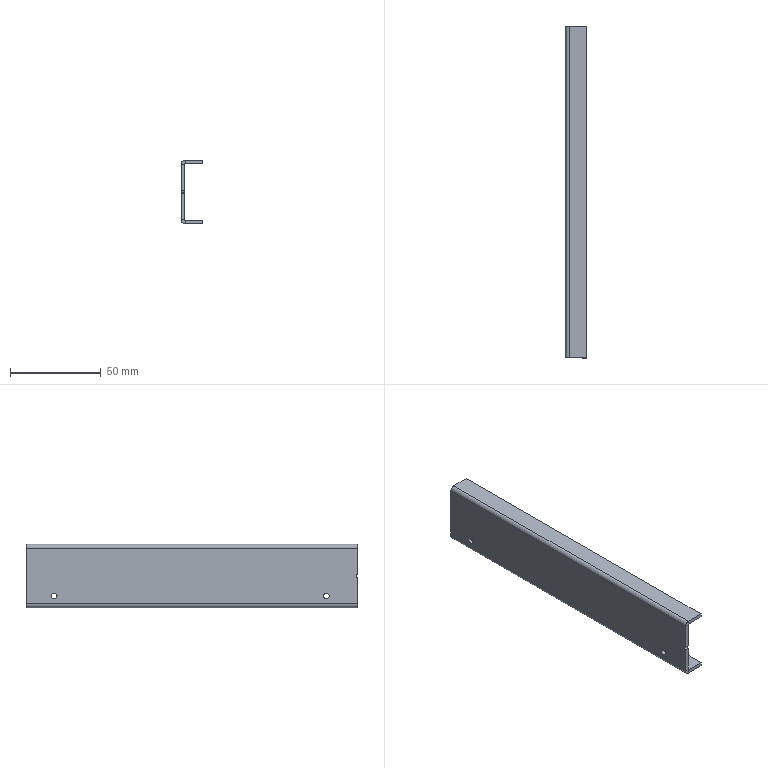Component | SolidWorks | PG50-06(BottomPlateWeldingDrawing)-1_BasePlateWeldment3-A(PG50-05-103-1 | 1 solid | 29 faces | box 12 x 183 x 35 mm | volume 19733 mm3 | plane 19 | cylinder 10 | commonest cylinder face diameters 3.2 x4 2 x2 4.3 x2 0.3 x2 | material AISI 1045 Steel, cold drawn
STEP:
#1=COLOUR_RGB('',0.7922,0.8196,0.9333);
#2=FILL_AREA_STYLE_COLOUR('',#1);
#3=FILL_AREA_STYLE('',(#2));
#4=SURFACE_STYLE_FILL_AREA(#3);
#5=SURFACE_SIDE_STYLE('',(#4));
#6=SURFACE_STYLE_USAGE(.BOTH.,#5);
#7=PRESENTATION_STYLE_ASSIGNMENT((#6));
#8=CARTESIAN_POINT('',(39.678,7.603,-4.154));
#9=VERTEX_POINT('',#8);
#10=CARTESIAN_POINT('',(39.678,7.729,-4.154));
#11=VERTEX_POINT('',#10);
#12=CARTESIAN_POINT('',(39.678,7.666,-4.154));
#13=DIRECTION('',(1.,-0.,0.));
#14=DIRECTION('',(0.,1.,0.));
#15=AXIS2_PLACEMENT_3D('',#12,#13,#14);
#16=CIRCLE('',#15,0.06299);
#17=EDGE_CURVE('',#9,#11,#16,.T.);
#18=ORIENTED_EDGE('',*,*,#17,.F.);
#19=CARTESIAN_POINT('',(39.757,7.603,-4.154));
#20=VERTEX_POINT('',#19);
#21=CARTESIAN_POINT('',(39.678,7.603,-4.154));
#22=DIRECTION('',(1.,-0.,0.));
#23=VECTOR('',#22,39.37);
#24=LINE('',#21,#23);
#25=EDGE_CURVE('',#9,#20,#24,.T.);
#26=ORIENTED_EDGE('',*,*,#25,.T.);
#27=CARTESIAN_POINT('',(39.757,7.729,-4.154));
#28=VERTEX_POINT('',#27);
#29=CARTESIAN_POINT('',(39.757,7.666,-4.154));
#30=DIRECTION('',(1.,-0.,0.));
#31=DIRECTION('',(0.,1.,0.));
#32=AXIS2_PLACEMENT_3D('',#29,#30,#31);
#33=CIRCLE('',#32,0.06299);
#34=EDGE_CURVE('',#20,#28,#33,.T.);
#35=ORIENTED_EDGE('',*,*,#34,.T.);
#36=CARTESIAN_POINT('',(39.678,7.729,-4.154));
#37=DIRECTION('',(1.,-0.,0.));
#38=VECTOR('',#37,39.37);
#39=LINE('',#36,#38);
#40=EDGE_CURVE('',#11,#28,#39,.T.);
#41=ORIENTED_EDGE('',*,*,#40,.F.);
#42=EDGE_LOOP('',(#18,#26,#35,#41));
#43=FACE_OUTER_BOUND('',#42,.T.);
#44=CARTESIAN_POINT('',(39.678,7.666,-4.154));
#45=DIRECTION('',(1.,-0.,0.));
#46=DIRECTION('',(0.,1.,0.));
#47=AXIS2_PLACEMENT_3D('',#44,#45,#46);
#48=CYLINDRICAL_SURFACE('',#47,0.06299);
#49=ADVANCED_FACE('',(#43),#48,.F.);
#50=CARTESIAN_POINT('',(39.678,1.697,-4.154));
#51=VERTEX_POINT('',#50);
#52=CARTESIAN_POINT('',(39.678,1.823,-4.154));
#53=VERTEX_POINT('',#52);
#54=CARTESIAN_POINT('',(39.678,1.76,-4.154));
#55=DIRECTION('',(1.,-0.,0.));
#56=DIRECTION('',(0.,1.,0.));
#57=AXIS2_PLACEMENT_3D('',#54,#55,#56);
#58=CIRCLE('',#57,0.06299);
#59=EDGE_CURVE('',#51,#53,#58,.T.);
#60=ORIENTED_EDGE('',*,*,#59,.F.);
#61=CARTESIAN_POINT('',(39.757,1.697,-4.154));
#62=VERTEX_POINT('',#61);
#63=CARTESIAN_POINT('',(39.678,1.697,-4.154));
#64=DIRECTION('',(1.,-0.,0.));
#65=VECTOR('',#64,39.37);
#66=LINE('',#63,#65);
#67=EDGE_CURVE('',#51,#62,#66,.T.);
#68=ORIENTED_EDGE('',*,*,#67,.T.);
#69=CARTESIAN_POINT('',(39.757,1.823,-4.154));
#70=VERTEX_POINT('',#69);
#71=CARTESIAN_POINT('',(39.757,1.76,-4.154));
#72=DIRECTION('',(1.,-0.,0.));
#73=DIRECTION('',(0.,1.,0.));
#74=AXIS2_PLACEMENT_3D('',#71,#72,#73);
#75=CIRCLE('',#74,0.06299);
#76=EDGE_CURVE('',#62,#70,#75,.T.);
#77=ORIENTED_EDGE('',*,*,#76,.T.);
#78=CARTESIAN_POINT('',(39.678,1.823,-4.154));
#79=DIRECTION('',(1.,-0.,0.));
#80=VECTOR('',#79,39.37);
#81=LINE('',#78,#80);
#82=EDGE_CURVE('',#53,#70,#81,.T.);
#83=ORIENTED_EDGE('',*,*,#82,.F.);
#84=EDGE_LOOP('',(#60,#68,#77,#83));
#85=FACE_OUTER_BOUND('',#84,.T.);
#86=CARTESIAN_POINT('',(39.678,1.76,-4.154));
#87=DIRECTION('',(1.,-0.,0.));
#88=DIRECTION('',(0.,1.,0.));
#89=AXIS2_PLACEMENT_3D('',#86,#87,#88);
#90=CYLINDRICAL_SURFACE('',#89,0.06299);
#91=ADVANCED_FACE('',(#85),#90,.F.);
#92=CARTESIAN_POINT('',(39.678,1.071,-3.681));
#93=VERTEX_POINT('',#92);
#94=CARTESIAN_POINT('',(39.678,1.11,-3.72));
#95=VERTEX_POINT('',#94);
#96=CARTESIAN_POINT('',(39.678,1.071,-3.72));
#97=DIRECTION('',(-1.,0.,-0.));
#98=DIRECTION('',(0.,1.,0.));
#99=AXIS2_PLACEMENT_3D('',#96,#97,#98);
#100=CIRCLE('',#99,0.03937);
#101=EDGE_CURVE('',#93,#95,#100,.T.);
#102=ORIENTED_EDGE('',*,*,#101,.T.);
#103=CARTESIAN_POINT('',(39.757,1.11,-3.72));
#104=VERTEX_POINT('',#103);
#105=CARTESIAN_POINT('',(39.678,1.11,-3.72));
#106=DIRECTION('',(1.,-0.,0.));
#107=VECTOR('',#106,39.37);
#108=LINE('',#105,#107);
#109=EDGE_CURVE('',#95,#104,#108,.T.);
#110=ORIENTED_EDGE('',*,*,#109,.T.);
#111=CARTESIAN_POINT('',(39.757,1.071,-3.681));
#112=VERTEX_POINT('',#111);
#113=CARTESIAN_POINT('',(39.757,1.071,-3.72));
#114=DIRECTION('',(-1.,0.,-0.));
#115=DIRECTION('',(0.,1.,0.));
#116=AXIS2_PLACEMENT_3D('',#113,#114,#115);
#117=CIRCLE('',#116,0.03937);
#118=EDGE_CURVE('',#112,#104,#117,.T.);
#119=ORIENTED_EDGE('',*,*,#118,.F.);
#120=CARTESIAN_POINT('',(39.678,1.071,-3.681));
#121=DIRECTION('',(1.,-0.,0.));
#122=VECTOR('',#121,39.37);
#123=LINE('',#120,#122);
#124=EDGE_CURVE('',#93,#112,#123,.T.);
#125=ORIENTED_EDGE('',*,*,#124,.F.);
#126=EDGE_LOOP('',(#102,#110,#119,#125));
#127=FACE_OUTER_BOUND('',#126,.T.);
#128=CARTESIAN_POINT('',(39.678,1.071,-3.72));
#129=DIRECTION('',(1.,-0.,0.));
#130=DIRECTION('',(0.,1.,0.));
#131=AXIS2_PLACEMENT_3D('',#128,#129,#130);
#132=CYLINDRICAL_SURFACE('',#131,0.03937);
#133=ADVANCED_FACE('',(#127),#132,.F.);
#134=CARTESIAN_POINT('',(39.678,7.666,-4.154));
#135=DIRECTION('',(1.,-0.,0.));
#136=DIRECTION('',(0.,1.,0.));
#137=AXIS2_PLACEMENT_3D('',#134,#135,#136);
#138=CIRCLE('',#137,0.06299);
#139=EDGE_CURVE('',#11,#9,#138,.T.);
#140=ORIENTED_EDGE('',*,*,#139,.T.);
#141=ORIENTED_EDGE('',*,*,#17,.T.);
#142=EDGE_LOOP('',(#140,#141));
#143=FACE_BOUND('',#142,.T.);
#144=CARTESIAN_POINT('',(39.678,1.76,-4.154));
#145=DIRECTION('',(1.,-0.,0.));
#146=DIRECTION('',(0.,1.,0.));
#147=AXIS2_PLACEMENT_3D('',#144,#145,#146);
#148=CIRCLE('',#147,0.06299);
#149=EDGE_CURVE('',#53,#51,#148,.T.);
#150=ORIENTED_EDGE('',*,*,#149,.T.);
#151=ORIENTED_EDGE('',*,*,#59,.T.);
#152=EDGE_LOOP('',(#150,#151));
#153=FACE_BOUND('',#152,.T.);
#154=CARTESIAN_POINT('',(39.678,1.071,-3.116));
#155=VERTEX_POINT('',#154);
#156=CARTESIAN_POINT('',(39.678,8.276,-3.116));
#157=VERTEX_POINT('',#156);
#158=CARTESIAN_POINT('',(39.678,1.071,-3.116));
#159=DIRECTION('',(0.,1.,-0.));
#160=VECTOR('',#159,39.37);
#161=LINE('',#158,#160);
#162=EDGE_CURVE('',#155,#157,#161,.T.);
#163=ORIENTED_EDGE('',*,*,#162,.T.);
#164=CARTESIAN_POINT('',(39.678,8.276,-4.325));
#165=VERTEX_POINT('',#164);
#166=CARTESIAN_POINT('',(39.678,8.276,-4.409));
#167=DIRECTION('',(-0.,0.,1.));
#168=VECTOR('',#167,39.37);
#169=LINE('',#166,#168);
#170=EDGE_CURVE('',#165,#157,#169,.T.);
#171=ORIENTED_EDGE('',*,*,#170,.F.);
#172=CARTESIAN_POINT('',(39.678,1.071,-4.325));
#173=VERTEX_POINT('',#172);
#174=CARTESIAN_POINT('',(39.678,8.276,-4.325));
#175=DIRECTION('',(-0.,-1.,0.));
#176=VECTOR('',#175,39.37);
#177=LINE('',#174,#176);
#178=EDGE_CURVE('',#165,#173,#177,.T.);
#179=ORIENTED_EDGE('',*,*,#178,.T.);
#180=CARTESIAN_POINT('',(39.678,1.071,-3.76));
#181=VERTEX_POINT('',#180);
#182=CARTESIAN_POINT('',(39.678,1.071,-4.409));
#183=DIRECTION('',(0.,-0.,-1.));
#184=VECTOR('',#183,39.37);
#185=LINE('',#182,#184);
#186=EDGE_CURVE('',#181,#173,#185,.T.);
#187=ORIENTED_EDGE('',*,*,#186,.F.);
#188=CARTESIAN_POINT('',(39.678,1.071,-3.72));
#189=DIRECTION('',(-1.,0.,-0.));
#190=DIRECTION('',(0.,1.,0.));
#191=AXIS2_PLACEMENT_3D('',#188,#189,#190);
#192=CIRCLE('',#191,0.03937);
#193=EDGE_CURVE('',#95,#181,#192,.T.);
#194=ORIENTED_EDGE('',*,*,#193,.F.);
#195=ORIENTED_EDGE('',*,*,#101,.F.);
#196=CARTESIAN_POINT('',(39.678,1.071,-3.681));
#197=DIRECTION('',(0.,-0.,-1.));
#198=VECTOR('',#197,39.37);
#199=LINE('',#196,#198);
#200=EDGE_CURVE('',#155,#93,#199,.T.);
#201=ORIENTED_EDGE('',*,*,#200,.F.);
#202=EDGE_LOOP('',(#163,#171,#179,#187,#194,#195,#201));
#203=FACE_OUTER_BOUND('',#202,.T.);
#204=CARTESIAN_POINT('',(39.678,1.071,-3.72));
#205=DIRECTION('',(1.,-0.,0.));
#206=DIRECTION('',(0.,1.,-0.));
#207=AXIS2_PLACEMENT_3D('',#204,#205,#206);
#208=PLANE('',#207);
#209=ADVANCED_FACE('',(#143,#153,#203),#208,.F.);
#210=CARTESIAN_POINT('',(39.757,7.666,-4.154));
#211=DIRECTION('',(1.,-0.,0.));
#212=DIRECTION('',(0.,1.,0.));
#213=AXIS2_PLACEMENT_3D('',#210,#211,#212);
#214=CIRCLE('',#213,0.06299);
#215=EDGE_CURVE('',#28,#20,#214,.T.);
#216=ORIENTED_EDGE('',*,*,#215,.F.);
#217=ORIENTED_EDGE('',*,*,#34,.F.);
#218=EDGE_LOOP('',(#216,#217));
#219=FACE_BOUND('',#218,.T.);
#220=CARTESIAN_POINT('',(39.757,1.76,-4.154));
#221=DIRECTION('',(1.,-0.,0.));
#222=DIRECTION('',(0.,1.,0.));
#223=AXIS2_PLACEMENT_3D('',#220,#221,#222);
#224=CIRCLE('',#223,0.06299);
#225=EDGE_CURVE('',#70,#62,#224,.T.);
#226=ORIENTED_EDGE('',*,*,#225,.F.);
#227=ORIENTED_EDGE('',*,*,#76,.F.);
#228=EDGE_LOOP('',(#226,#227));
#229=FACE_BOUND('',#228,.T.);
#230=CARTESIAN_POINT('',(39.757,8.276,-4.325));
#231=VERTEX_POINT('',#230);
#232=CARTESIAN_POINT('',(39.757,8.276,-3.116));
#233=VERTEX_POINT('',#232);
#234=CARTESIAN_POINT('',(39.757,8.276,-4.409));
#235=DIRECTION('',(-0.,0.,1.));
#236=VECTOR('',#235,39.37);
#237=LINE('',#234,#236);
#238=EDGE_CURVE('',#231,#233,#237,.T.);
#239=ORIENTED_EDGE('',*,*,#238,.T.);
#240=CARTESIAN_POINT('',(39.757,1.071,-3.116));
#241=VERTEX_POINT('',#240);
#242=CARTESIAN_POINT('',(39.757,1.071,-3.116));
#243=DIRECTION('',(0.,1.,-0.));
#244=VECTOR('',#243,39.37);
#245=LINE('',#242,#244);
#246=EDGE_CURVE('',#241,#233,#245,.T.);
#247=ORIENTED_EDGE('',*,*,#246,.F.);
#248=CARTESIAN_POINT('',(39.757,1.071,-3.681));
#249=DIRECTION('',(0.,-0.,-1.));
#250=VECTOR('',#249,39.37);
#251=LINE('',#248,#250);
#252=EDGE_CURVE('',#241,#112,#251,.T.);
#253=ORIENTED_EDGE('',*,*,#252,.T.);
#254=ORIENTED_EDGE('',*,*,#118,.T.);
#255=CARTESIAN_POINT('',(39.757,1.071,-3.76));
#256=VERTEX_POINT('',#255);
#257=CARTESIAN_POINT('',(39.757,1.071,-3.72));
#258=DIRECTION('',(-1.,0.,-0.));
#259=DIRECTION('',(0.,1.,0.));
#260=AXIS2_PLACEMENT_3D('',#257,#258,#259);
#261=CIRCLE('',#260,0.03937);
#262=EDGE_CURVE('',#104,#256,#261,.T.);
#263=ORIENTED_EDGE('',*,*,#262,.T.);
#264=CARTESIAN_POINT('',(39.757,1.071,-4.325));
#265=VERTEX_POINT('',#264);
#266=CARTESIAN_POINT('',(39.757,1.071,-4.409));
#267=DIRECTION('',(0.,-0.,-1.));
#268=VECTOR('',#267,39.37);
#269=LINE('',#266,#268);
#270=EDGE_CURVE('',#256,#265,#269,.T.);
#271=ORIENTED_EDGE('',*,*,#270,.T.);
#272=CARTESIAN_POINT('',(39.757,8.276,-4.325));
#273=DIRECTION('',(-0.,-1.,0.));
#274=VECTOR('',#273,39.37);
#275=LINE('',#272,#274);
#276=EDGE_CURVE('',#231,#265,#275,.T.);
#277=ORIENTED_EDGE('',*,*,#276,.F.);
#278=EDGE_LOOP('',(#239,#247,#253,#254,#263,#271,#277));
#279=FACE_OUTER_BOUND('',#278,.T.);
#280=CARTESIAN_POINT('',(39.757,1.071,-3.72));
#281=DIRECTION('',(1.,-0.,0.));
#282=DIRECTION('',(0.,1.,-0.));
#283=AXIS2_PLACEMENT_3D('',#280,#281,#282);
#284=PLANE('',#283);
#285=ADVANCED_FACE('',(#219,#229,#279),#284,.T.);
#286=ORIENTED_EDGE('',*,*,#252,.F.);
#287=CARTESIAN_POINT('',(39.757,1.071,-3.116));
#288=DIRECTION('',(-1.,0.,-0.));
#289=VECTOR('',#288,39.37);
#290=LINE('',#287,#289);
#291=EDGE_CURVE('',#241,#155,#290,.T.);
#292=ORIENTED_EDGE('',*,*,#291,.T.);
#293=ORIENTED_EDGE('',*,*,#200,.T.);
#294=ORIENTED_EDGE('',*,*,#124,.T.);
#295=EDGE_LOOP('',(#286,#292,#293,#294));
#296=FACE_OUTER_BOUND('',#295,.T.);
#297=CARTESIAN_POINT('',(39.678,1.071,-3.681));
#298=DIRECTION('',(-0.,-1.,0.));
#299=DIRECTION('',(1.,-0.,0.));
#300=AXIS2_PLACEMENT_3D('',#297,#298,#299);
#301=PLANE('',#300);
#302=ADVANCED_FACE('',(#296),#301,.T.);
#303=CARTESIAN_POINT('',(39.757,8.276,-3.116));
#304=DIRECTION('',(-1.,0.,-0.));
#305=VECTOR('',#304,39.37);
#306=LINE('',#303,#305);
#307=EDGE_CURVE('',#233,#157,#306,.T.);
#308=ORIENTED_EDGE('',*,*,#307,.F.);
#309=ORIENTED_EDGE('',*,*,#238,.F.);
#310=CARTESIAN_POINT('',(39.757,8.276,-4.325));
#311=DIRECTION('',(-1.,0.,-0.));
#312=VECTOR('',#311,39.37);
#313=LINE('',#310,#312);
#314=EDGE_CURVE('',#231,#165,#313,.T.);
#315=ORIENTED_EDGE('',*,*,#314,.T.);
#316=ORIENTED_EDGE('',*,*,#170,.T.);
#317=EDGE_LOOP('',(#308,#309,#315,#316));
#318=FACE_OUTER_BOUND('',#317,.T.);
#319=CARTESIAN_POINT('',(39.678,8.276,-4.409));
#320=DIRECTION('',(0.,1.,-0.));
#321=DIRECTION('',(-1.,0.,-0.));
#322=AXIS2_PLACEMENT_3D('',#319,#320,#321);
#323=PLANE('',#322);
#324=ADVANCED_FACE('',(#318),#323,.T.);
#325=CARTESIAN_POINT('',(39.757,1.071,-4.325));
#326=DIRECTION('',(-1.,0.,-0.));
#327=VECTOR('',#326,39.37);
#328=LINE('',#325,#327);
#329=EDGE_CURVE('',#265,#173,#328,.T.);
#330=ORIENTED_EDGE('',*,*,#329,.F.);
#331=ORIENTED_EDGE('',*,*,#270,.F.);
#332=CARTESIAN_POINT('',(39.678,1.071,-3.76));
#333=DIRECTION('',(1.,-0.,0.));
#334=VECTOR('',#333,39.37);
#335=LINE('',#332,#334);
#336=EDGE_CURVE('',#181,#256,#335,.T.);
#337=ORIENTED_EDGE('',*,*,#336,.F.);
#338=ORIENTED_EDGE('',*,*,#186,.T.);
#339=EDGE_LOOP('',(#330,#331,#337,#338));
#340=FACE_OUTER_BOUND('',#339,.T.);
#341=CARTESIAN_POINT('',(39.678,1.071,-4.409));
#342=DIRECTION('',(-0.,-1.,0.));
#343=DIRECTION('',(1.,-0.,0.));
#344=AXIS2_PLACEMENT_3D('',#341,#342,#343);
#345=PLANE('',#344);
#346=ADVANCED_FACE('',(#340),#345,.T.);
#347=ORIENTED_EDGE('',*,*,#109,.F.);
#348=ORIENTED_EDGE('',*,*,#193,.T.);
#349=ORIENTED_EDGE('',*,*,#336,.T.);
#350=ORIENTED_EDGE('',*,*,#262,.F.);
#351=EDGE_LOOP('',(#347,#348,#349,#350));
#352=FACE_OUTER_BOUND('',#351,.T.);
#353=CARTESIAN_POINT('',(39.678,1.071,-3.72));
#354=DIRECTION('',(1.,-0.,0.));
#355=DIRECTION('',(0.,1.,0.));
#356=AXIS2_PLACEMENT_3D('',#353,#354,#355);
#357=CYLINDRICAL_SURFACE('',#356,0.03937);
#358=ADVANCED_FACE('',(#352),#357,.F.);
#359=ORIENTED_EDGE('',*,*,#67,.F.);
#360=ORIENTED_EDGE('',*,*,#149,.F.);
#361=ORIENTED_EDGE('',*,*,#82,.T.);
#362=ORIENTED_EDGE('',*,*,#225,.T.);
#363=EDGE_LOOP('',(#359,#360,#361,#362));
#364=FACE_OUTER_BOUND('',#363,.T.);
#365=CARTESIAN_POINT('',(39.678,1.76,-4.154));
#366=DIRECTION('',(1.,-0.,0.));
#367=DIRECTION('',(0.,1.,0.));
#368=AXIS2_PLACEMENT_3D('',#365,#366,#367);
#369=CYLINDRICAL_SURFACE('',#368,0.06299);
#370=ADVANCED_FACE('',(#364),#369,.F.);
#371=ORIENTED_EDGE('',*,*,#25,.F.);
#372=ORIENTED_EDGE('',*,*,#139,.F.);
#373=ORIENTED_EDGE('',*,*,#40,.T.);
#374=ORIENTED_EDGE('',*,*,#215,.T.);
#375=EDGE_LOOP('',(#371,#372,#373,#374));
#376=FACE_OUTER_BOUND('',#375,.T.);
#377=CARTESIAN_POINT('',(39.678,7.666,-4.154));
#378=DIRECTION('',(1.,-0.,0.));
#379=DIRECTION('',(0.,1.,0.));
#380=AXIS2_PLACEMENT_3D('',#377,#378,#379);
#381=CYLINDRICAL_SURFACE('',#380,0.06299);
#382=ADVANCED_FACE('',(#376),#381,.F.);
#383=CARTESIAN_POINT('',(39.763,1.071,-4.331));
#384=VERTEX_POINT('',#383);
#385=CARTESIAN_POINT('',(39.763,1.071,-4.409));
#386=VERTEX_POINT('',#385);
#387=CARTESIAN_POINT('',(39.763,1.071,-4.409));
#388=DIRECTION('',(-0.,-0.,-1.));
#389=VECTOR('',#388,39.37);
#390=LINE('',#387,#389);
#391=EDGE_CURVE('',#384,#386,#390,.T.);
#392=ORIENTED_EDGE('',*,*,#391,.F.);
#393=CARTESIAN_POINT('',(39.763,1.071,-4.325));
#394=DIRECTION('',(-0.,-1.,0.));
#395=DIRECTION('',(-1.,0.,0.));
#396=AXIS2_PLACEMENT_3D('',#393,#394,#395);
#397=CIRCLE('',#396,0.005906);
#398=EDGE_CURVE('',#265,#384,#397,.T.);
#399=ORIENTED_EDGE('',*,*,#398,.F.);
#400=ORIENTED_EDGE('',*,*,#329,.T.);
#401=CARTESIAN_POINT('',(39.763,1.071,-4.325));
#402=DIRECTION('',(-0.,-1.,0.));
#403=DIRECTION('',(-1.,0.,0.));
#404=AXIS2_PLACEMENT_3D('',#401,#402,#403);
#405=CIRCLE('',#404,0.08465);
#406=EDGE_CURVE('',#173,#386,#405,.T.);
#407=ORIENTED_EDGE('',*,*,#406,.T.);
#408=EDGE_LOOP('',(#392,#399,#400,#407));
#409=FACE_OUTER_BOUND('',#408,.T.);
#410=CARTESIAN_POINT('',(39.763,1.071,-4.325));
#411=DIRECTION('',(-0.,-1.,0.));
#412=DIRECTION('',(1.,-0.,0.));
#413=AXIS2_PLACEMENT_3D('',#410,#411,#412);
#414=PLANE('',#413);
#415=ADVANCED_FACE('',(#409),#414,.T.);
#416=CARTESIAN_POINT('',(39.763,8.276,-4.331));
#417=VERTEX_POINT('',#416);
#418=CARTESIAN_POINT('',(39.763,8.276,-4.325));
#419=DIRECTION('',(0.,1.,-0.));
#420=DIRECTION('',(-1.,0.,0.));
#421=AXIS2_PLACEMENT_3D('',#418,#419,#420);
#422=CIRCLE('',#421,0.005906);
#423=EDGE_CURVE('',#417,#231,#422,.T.);
#424=ORIENTED_EDGE('',*,*,#423,.F.);
#425=CARTESIAN_POINT('',(39.763,8.276,-4.409));
#426=VERTEX_POINT('',#425);
#427=CARTESIAN_POINT('',(39.763,8.276,-4.331));
#428=DIRECTION('',(-0.,-0.,-1.));
#429=VECTOR('',#428,39.37);
#430=LINE('',#427,#429);
#431=EDGE_CURVE('',#417,#426,#430,.T.);
#432=ORIENTED_EDGE('',*,*,#431,.T.);
#433=CARTESIAN_POINT('',(39.763,8.276,-4.325));
#434=DIRECTION('',(0.,1.,-0.));
#435=DIRECTION('',(-1.,0.,0.));
#436=AXIS2_PLACEMENT_3D('',#433,#434,#435);
#437=CIRCLE('',#436,0.08465);
#438=EDGE_CURVE('',#426,#165,#437,.T.);
#439=ORIENTED_EDGE('',*,*,#438,.T.);
#440=ORIENTED_EDGE('',*,*,#314,.F.);
#441=EDGE_LOOP('',(#424,#432,#439,#440));
#442=FACE_OUTER_BOUND('',#441,.T.);
#443=CARTESIAN_POINT('',(39.763,8.276,-4.325));
#444=DIRECTION('',(-0.,-1.,0.));
#445=DIRECTION('',(1.,-0.,0.));
#446=AXIS2_PLACEMENT_3D('',#443,#444,#445);
#447=PLANE('',#446);
#448=ADVANCED_FACE('',(#442),#447,.F.);
#449=ORIENTED_EDGE('',*,*,#178,.F.);
#450=ORIENTED_EDGE('',*,*,#438,.F.);
#451=CARTESIAN_POINT('',(39.763,1.071,-4.409));
#452=DIRECTION('',(-0.,-1.,0.));
#453=VECTOR('',#452,39.37);
#454=LINE('',#451,#453);
#455=EDGE_CURVE('',#426,#386,#454,.T.);
#456=ORIENTED_EDGE('',*,*,#455,.T.);
#457=ORIENTED_EDGE('',*,*,#406,.F.);
#458=EDGE_LOOP('',(#449,#450,#456,#457));
#459=FACE_OUTER_BOUND('',#458,.T.);
#460=CARTESIAN_POINT('',(39.763,8.276,-4.325));
#461=DIRECTION('',(0.,1.,-0.));
#462=DIRECTION('',(0.,0.,-1.));
#463=AXIS2_PLACEMENT_3D('',#460,#461,#462);
#464=CYLINDRICAL_SURFACE('',#463,0.08465);
#465=ADVANCED_FACE('',(#459),#464,.T.);
#466=ORIENTED_EDGE('',*,*,#276,.T.);
#467=ORIENTED_EDGE('',*,*,#398,.T.);
#468=CARTESIAN_POINT('',(39.763,1.071,-4.331));
#469=DIRECTION('',(0.,1.,-0.));
#470=VECTOR('',#469,39.37);
#471=LINE('',#468,#470);
#472=EDGE_CURVE('',#384,#417,#471,.T.);
#473=ORIENTED_EDGE('',*,*,#472,.T.);
#474=ORIENTED_EDGE('',*,*,#423,.T.);
#475=EDGE_LOOP('',(#466,#467,#473,#474));
#476=FACE_OUTER_BOUND('',#475,.T.);
#477=CARTESIAN_POINT('',(39.763,8.276,-4.325));
#478=DIRECTION('',(0.,1.,-0.));
#479=DIRECTION('',(0.,0.,-1.));
#480=AXIS2_PLACEMENT_3D('',#477,#478,#479);
#481=CYLINDRICAL_SURFACE('',#480,0.005906);
#482=ADVANCED_FACE('',(#476),#481,.F.);
#483=ORIENTED_EDGE('',*,*,#391,.T.);
#484=CARTESIAN_POINT('',(40.15,1.071,-4.409));
#485=VERTEX_POINT('',#484);
#486=CARTESIAN_POINT('',(39.757,1.071,-4.409));
#487=DIRECTION('',(-1.,0.,0.));
#488=VECTOR('',#487,39.37);
#489=LINE('',#486,#488);
#490=EDGE_CURVE('',#485,#386,#489,.T.);
#491=ORIENTED_EDGE('',*,*,#490,.F.);
#492=CARTESIAN_POINT('',(40.15,1.071,-4.331));
#493=VERTEX_POINT('',#492);
#494=CARTESIAN_POINT('',(40.15,1.071,-4.409));
#495=DIRECTION('',(0.,0.,1.));
#496=VECTOR('',#495,39.37);
#497=LINE('',#494,#496);
#498=EDGE_CURVE('',#485,#493,#497,.T.);
#499=ORIENTED_EDGE('',*,*,#498,.T.);
#500=CARTESIAN_POINT('',(39.757,1.071,-4.331));
#501=DIRECTION('',(-1.,0.,0.));
#502=VECTOR('',#501,39.37);
#503=LINE('',#500,#502);
#504=EDGE_CURVE('',#493,#384,#503,.T.);
#505=ORIENTED_EDGE('',*,*,#504,.T.);
#506=EDGE_LOOP('',(#483,#491,#499,#505));
#507=FACE_OUTER_BOUND('',#506,.T.);
#508=CARTESIAN_POINT('',(39.757,1.071,-4.409));
#509=DIRECTION('',(0.,1.,-0.));
#510=DIRECTION('',(-1.,0.,-0.));
#511=AXIS2_PLACEMENT_3D('',#508,#509,#510);
#512=PLANE('',#511);
#513=ADVANCED_FACE('',(#507),#512,.F.);
#514=ORIENTED_EDGE('',*,*,#431,.F.);
#515=CARTESIAN_POINT('',(40.15,8.276,-4.331));
#516=VERTEX_POINT('',#515);
#517=CARTESIAN_POINT('',(40.15,8.276,-4.331));
#518=DIRECTION('',(1.,-0.,-0.));
#519=VECTOR('',#518,39.37);
#520=LINE('',#517,#519);
#521=EDGE_CURVE('',#417,#516,#520,.T.);
#522=ORIENTED_EDGE('',*,*,#521,.T.);
#523=CARTESIAN_POINT('',(40.15,8.276,-4.409));
#524=VERTEX_POINT('',#523);
#525=CARTESIAN_POINT('',(40.15,8.276,-4.409));
#526=DIRECTION('',(0.,0.,1.));
#527=VECTOR('',#526,39.37);
#528=LINE('',#525,#527);
#529=EDGE_CURVE('',#524,#516,#528,.T.);
#530=ORIENTED_EDGE('',*,*,#529,.F.);
#531=CARTESIAN_POINT('',(39.757,8.276,-4.409));
#532=DIRECTION('',(1.,-0.,-0.));
#533=VECTOR('',#532,39.37);
#534=LINE('',#531,#533);
#535=EDGE_CURVE('',#426,#524,#534,.T.);
#536=ORIENTED_EDGE('',*,*,#535,.F.);
#537=EDGE_LOOP('',(#514,#522,#530,#536));
#538=FACE_OUTER_BOUND('',#537,.T.);
#539=CARTESIAN_POINT('',(40.15,8.276,-4.409));
#540=DIRECTION('',(-0.,-1.,0.));
#541=DIRECTION('',(1.,-0.,0.));
#542=AXIS2_PLACEMENT_3D('',#539,#540,#541);
#543=PLANE('',#542);
#544=ADVANCED_FACE('',(#538),#543,.F.);
#545=ORIENTED_EDGE('',*,*,#455,.F.);
#546=ORIENTED_EDGE('',*,*,#535,.T.);
#547=CARTESIAN_POINT('',(40.15,4.673,-4.409));
#548=DIRECTION('',(-0.,-1.,0.));
#549=VECTOR('',#548,39.37);
#550=LINE('',#547,#549);
#551=EDGE_CURVE('',#524,#485,#550,.T.);
#552=ORIENTED_EDGE('',*,*,#551,.T.);
#553=ORIENTED_EDGE('',*,*,#490,.T.);
#554=EDGE_LOOP('',(#545,#546,#552,#553));
#555=FACE_OUTER_BOUND('',#554,.T.);
#556=CARTESIAN_POINT('',(39.757,4.673,-4.409));
#557=DIRECTION('',(0.,0.,1.));
#558=DIRECTION('',(1.,-0.,-0.));
#559=AXIS2_PLACEMENT_3D('',#556,#557,#558);
#560=PLANE('',#559);
#561=ADVANCED_FACE('',(#555),#560,.F.);
#562=ORIENTED_EDGE('',*,*,#521,.F.);
#563=ORIENTED_EDGE('',*,*,#472,.F.);
#564=ORIENTED_EDGE('',*,*,#504,.F.);
#565=CARTESIAN_POINT('',(40.15,1.071,-4.331));
#566=DIRECTION('',(-0.,-1.,0.));
#567=VECTOR('',#566,39.37);
#568=LINE('',#565,#567);
#569=EDGE_CURVE('',#516,#493,#568,.T.);
#570=ORIENTED_EDGE('',*,*,#569,.F.);
#571=EDGE_LOOP('',(#562,#563,#564,#570));
#572=FACE_OUTER_BOUND('',#571,.T.);
#573=CARTESIAN_POINT('',(39.757,4.673,-4.331));
#574=DIRECTION('',(0.,0.,1.));
#575=DIRECTION('',(1.,-0.,-0.));
#576=AXIS2_PLACEMENT_3D('',#573,#574,#575);
#577=PLANE('',#576);
#578=ADVANCED_FACE('',(#572),#577,.T.);
#579=ORIENTED_EDGE('',*,*,#569,.T.);
#580=ORIENTED_EDGE('',*,*,#498,.F.);
#581=ORIENTED_EDGE('',*,*,#551,.F.);
#582=ORIENTED_EDGE('',*,*,#529,.T.);
#583=EDGE_LOOP('',(#579,#580,#581,#582));
#584=FACE_OUTER_BOUND('',#583,.T.);
#585=CARTESIAN_POINT('',(40.15,1.071,-4.409));
#586=DIRECTION('',(-1.,0.,0.));
#587=DIRECTION('',(0.,0.,1.));
#588=AXIS2_PLACEMENT_3D('',#585,#586,#587);
#589=PLANE('',#588);
#590=ADVANCED_FACE('',(#584),#589,.F.);
#591=CARTESIAN_POINT('',(39.763,8.276,-3.11));
#592=VERTEX_POINT('',#591);
#593=CARTESIAN_POINT('',(39.763,8.276,-3.031));
#594=VERTEX_POINT('',#593);
#595=CARTESIAN_POINT('',(39.763,8.276,-3.031));
#596=DIRECTION('',(-0.,0.,1.));
#597=VECTOR('',#596,39.37);
#598=LINE('',#595,#597);
#599=EDGE_CURVE('',#592,#594,#598,.T.);
#600=ORIENTED_EDGE('',*,*,#599,.F.);
#601=CARTESIAN_POINT('',(39.763,8.276,-3.116));
#602=DIRECTION('',(0.,1.,-0.));
#603=DIRECTION('',(1.,0.,0.));
#604=AXIS2_PLACEMENT_3D('',#601,#602,#603);
#605=CIRCLE('',#604,0.005906);
#606=EDGE_CURVE('',#233,#592,#605,.T.);
#607=ORIENTED_EDGE('',*,*,#606,.F.);
#608=ORIENTED_EDGE('',*,*,#307,.T.);
#609=CARTESIAN_POINT('',(39.763,8.276,-3.116));
#610=DIRECTION('',(0.,1.,-0.));
#611=DIRECTION('',(1.,0.,0.));
#612=AXIS2_PLACEMENT_3D('',#609,#610,#611);
#613=CIRCLE('',#612,0.08465);
#614=EDGE_CURVE('',#157,#594,#613,.T.);
#615=ORIENTED_EDGE('',*,*,#614,.T.);
#616=EDGE_LOOP('',(#600,#607,#608,#615));
#617=FACE_OUTER_BOUND('',#616,.T.);
#618=CARTESIAN_POINT('',(39.763,8.276,-3.116));
#619=DIRECTION('',(0.,1.,-0.));
#620=DIRECTION('',(-1.,0.,-0.));
#621=AXIS2_PLACEMENT_3D('',#618,#619,#620);
#622=PLANE('',#621);
#623=ADVANCED_FACE('',(#617),#622,.T.);
#624=CARTESIAN_POINT('',(39.763,1.071,-3.11));
#625=VERTEX_POINT('',#624);
#626=CARTESIAN_POINT('',(39.763,1.071,-3.116));
#627=DIRECTION('',(-0.,-1.,0.));
#628=DIRECTION('',(1.,0.,0.));
#629=AXIS2_PLACEMENT_3D('',#626,#627,#628);
#630=CIRCLE('',#629,0.005906);
#631=EDGE_CURVE('',#625,#241,#630,.T.);
#632=ORIENTED_EDGE('',*,*,#631,.F.);
#633=CARTESIAN_POINT('',(39.763,1.071,-3.031));
#634=VERTEX_POINT('',#633);
#635=CARTESIAN_POINT('',(39.763,1.071,-3.11));
#636=DIRECTION('',(-0.,0.,1.));
#637=VECTOR('',#636,39.37);
#638=LINE('',#635,#637);
#639=EDGE_CURVE('',#625,#634,#638,.T.);
#640=ORIENTED_EDGE('',*,*,#639,.T.);
#641=CARTESIAN_POINT('',(39.763,1.071,-3.116));
#642=DIRECTION('',(-0.,-1.,0.));
#643=DIRECTION('',(1.,-0.,0.));
#644=AXIS2_PLACEMENT_3D('',#641,#642,#643);
#645=CIRCLE('',#644,0.08465);
#646=EDGE_CURVE('',#634,#155,#645,.T.);
#647=ORIENTED_EDGE('',*,*,#646,.T.);
#648=ORIENTED_EDGE('',*,*,#291,.F.);
#649=EDGE_LOOP('',(#632,#640,#647,#648));
#650=FACE_OUTER_BOUND('',#649,.T.);
#651=CARTESIAN_POINT('',(39.763,1.071,-3.116));
#652=DIRECTION('',(0.,1.,-0.));
#653=DIRECTION('',(-1.,0.,-0.));
#654=AXIS2_PLACEMENT_3D('',#651,#652,#653);
#655=PLANE('',#654);
#656=ADVANCED_FACE('',(#650),#655,.F.);
#657=ORIENTED_EDGE('',*,*,#162,.F.);
#658=ORIENTED_EDGE('',*,*,#646,.F.);
#659=CARTESIAN_POINT('',(39.763,8.276,-3.031));
#660=DIRECTION('',(0.,1.,-0.));
#661=VECTOR('',#660,39.37);
#662=LINE('',#659,#661);
#663=EDGE_CURVE('',#634,#594,#662,.T.);
#664=ORIENTED_EDGE('',*,*,#663,.T.);
#665=ORIENTED_EDGE('',*,*,#614,.F.);
#666=EDGE_LOOP('',(#657,#658,#664,#665));
#667=FACE_OUTER_BOUND('',#666,.T.);
#668=CARTESIAN_POINT('',(39.763,1.071,-3.116));
#669=DIRECTION('',(-0.,-1.,0.));
#670=DIRECTION('',(0.,0.,1.));
#671=AXIS2_PLACEMENT_3D('',#668,#669,#670);
#672=CYLINDRICAL_SURFACE('',#671,0.08465);
#673=ADVANCED_FACE('',(#667),#672,.T.);
#674=ORIENTED_EDGE('',*,*,#246,.T.);
#675=ORIENTED_EDGE('',*,*,#606,.T.);
#676=CARTESIAN_POINT('',(39.763,8.276,-3.11));
#677=DIRECTION('',(-0.,-1.,0.));
#678=VECTOR('',#677,39.37);
#679=LINE('',#676,#678);
#680=EDGE_CURVE('',#592,#625,#679,.T.);
#681=ORIENTED_EDGE('',*,*,#680,.T.);
#682=ORIENTED_EDGE('',*,*,#631,.T.);
#683=EDGE_LOOP('',(#674,#675,#681,#682));
#684=FACE_OUTER_BOUND('',#683,.T.);
#685=CARTESIAN_POINT('',(39.763,1.071,-3.116));
#686=DIRECTION('',(-0.,-1.,0.));
#687=DIRECTION('',(0.,0.,1.));
#688=AXIS2_PLACEMENT_3D('',#685,#686,#687);
#689=CYLINDRICAL_SURFACE('',#688,0.005906);
#690=ADVANCED_FACE('',(#684),#689,.F.);
#691=ORIENTED_EDGE('',*,*,#639,.F.);
#692=CARTESIAN_POINT('',(40.15,1.071,-3.11));
#693=VERTEX_POINT('',#692);
#694=CARTESIAN_POINT('',(40.15,1.071,-3.11));
#695=DIRECTION('',(1.,-0.,0.));
#696=VECTOR('',#695,39.37);
#697=LINE('',#694,#696);
#698=EDGE_CURVE('',#625,#693,#697,.T.);
#699=ORIENTED_EDGE('',*,*,#698,.T.);
#700=CARTESIAN_POINT('',(40.15,1.071,-3.031));
#701=VERTEX_POINT('',#700);
#702=CARTESIAN_POINT('',(40.15,1.071,-3.031));
#703=DIRECTION('',(0.,-0.,-1.));
#704=VECTOR('',#703,39.37);
#705=LINE('',#702,#704);
#706=EDGE_CURVE('',#701,#693,#705,.T.);
#707=ORIENTED_EDGE('',*,*,#706,.F.);
#708=CARTESIAN_POINT('',(39.757,1.071,-3.031));
#709=DIRECTION('',(1.,-0.,0.));
#710=VECTOR('',#709,39.37);
#711=LINE('',#708,#710);
#712=EDGE_CURVE('',#634,#701,#711,.T.);
#713=ORIENTED_EDGE('',*,*,#712,.F.);
#714=EDGE_LOOP('',(#691,#699,#707,#713));
#715=FACE_OUTER_BOUND('',#714,.T.);
#716=CARTESIAN_POINT('',(40.15,1.071,-3.031));
#717=DIRECTION('',(0.,1.,-0.));
#718=DIRECTION('',(-1.,0.,-0.));
#719=AXIS2_PLACEMENT_3D('',#716,#717,#718);
#720=PLANE('',#719);
#721=ADVANCED_FACE('',(#715),#720,.F.);
#722=ORIENTED_EDGE('',*,*,#599,.T.);
#723=CARTESIAN_POINT('',(40.15,8.276,-3.031));
#724=VERTEX_POINT('',#723);
#725=CARTESIAN_POINT('',(39.757,8.276,-3.031));
#726=DIRECTION('',(-1.,0.,-0.));
#727=VECTOR('',#726,39.37);
#728=LINE('',#725,#727);
#729=EDGE_CURVE('',#724,#594,#728,.T.);
#730=ORIENTED_EDGE('',*,*,#729,.F.);
#731=CARTESIAN_POINT('',(40.15,8.276,-3.11));
#732=VERTEX_POINT('',#731);
#733=CARTESIAN_POINT('',(40.15,8.276,-3.031));
#734=DIRECTION('',(0.,-0.,-1.));
#735=VECTOR('',#734,39.37);
#736=LINE('',#733,#735);
#737=EDGE_CURVE('',#724,#732,#736,.T.);
#738=ORIENTED_EDGE('',*,*,#737,.T.);
#739=CARTESIAN_POINT('',(39.757,8.276,-3.11));
#740=DIRECTION('',(-1.,0.,-0.));
#741=VECTOR('',#740,39.37);
#742=LINE('',#739,#741);
#743=EDGE_CURVE('',#732,#592,#742,.T.);
#744=ORIENTED_EDGE('',*,*,#743,.T.);
#745=EDGE_LOOP('',(#722,#730,#738,#744));
#746=FACE_OUTER_BOUND('',#745,.T.);
#747=CARTESIAN_POINT('',(39.757,8.276,-3.031));
#748=DIRECTION('',(-0.,-1.,0.));
#749=DIRECTION('',(1.,-0.,0.));
#750=AXIS2_PLACEMENT_3D('',#747,#748,#749);
#751=PLANE('',#750);
#752=ADVANCED_FACE('',(#746),#751,.F.);
#753=ORIENTED_EDGE('',*,*,#663,.F.);
#754=ORIENTED_EDGE('',*,*,#712,.T.);
#755=CARTESIAN_POINT('',(40.15,4.673,-3.031));
#756=DIRECTION('',(0.,1.,-0.));
#757=VECTOR('',#756,39.37);
#758=LINE('',#755,#757);
#759=EDGE_CURVE('',#701,#724,#758,.T.);
#760=ORIENTED_EDGE('',*,*,#759,.T.);
#761=ORIENTED_EDGE('',*,*,#729,.T.);
#762=EDGE_LOOP('',(#753,#754,#760,#761));
#763=FACE_OUTER_BOUND('',#762,.T.);
#764=CARTESIAN_POINT('',(39.757,4.673,-3.031));
#765=DIRECTION('',(0.,-0.,-1.));
#766=DIRECTION('',(-1.,0.,-0.));
#767=AXIS2_PLACEMENT_3D('',#764,#765,#766);
#768=PLANE('',#767);
#769=ADVANCED_FACE('',(#763),#768,.F.);
#770=ORIENTED_EDGE('',*,*,#698,.F.);
#771=ORIENTED_EDGE('',*,*,#680,.F.);
#772=ORIENTED_EDGE('',*,*,#743,.F.);
#773=CARTESIAN_POINT('',(40.15,8.276,-3.11));
#774=DIRECTION('',(0.,1.,-0.));
#775=VECTOR('',#774,39.37);
#776=LINE('',#773,#775);
#777=EDGE_CURVE('',#693,#732,#776,.T.);
#778=ORIENTED_EDGE('',*,*,#777,.F.);
#779=EDGE_LOOP('',(#770,#771,#772,#778));
#780=FACE_OUTER_BOUND('',#779,.T.);
#781=CARTESIAN_POINT('',(39.757,4.673,-3.11));
#782=DIRECTION('',(0.,-0.,-1.));
#783=DIRECTION('',(-1.,0.,-0.));
#784=AXIS2_PLACEMENT_3D('',#781,#782,#783);
#785=PLANE('',#784);
#786=ADVANCED_FACE('',(#780),#785,.T.);
#787=ORIENTED_EDGE('',*,*,#777,.T.);
#788=ORIENTED_EDGE('',*,*,#737,.F.);
#789=ORIENTED_EDGE('',*,*,#759,.F.);
#790=ORIENTED_EDGE('',*,*,#706,.T.);
#791=EDGE_LOOP('',(#787,#788,#789,#790));
#792=FACE_OUTER_BOUND('',#791,.T.);
#793=CARTESIAN_POINT('',(40.15,8.276,-3.031));
#794=DIRECTION('',(-1.,0.,-0.));
#795=DIRECTION('',(-0.,0.,1.));
#796=AXIS2_PLACEMENT_3D('',#793,#794,#795);
#797=PLANE('',#796);
#798=ADVANCED_FACE('',(#792),#797,.F.);
#799=CLOSED_SHELL('',(#49,#91,#133,#209,#285,#302,#324,#346,#358,#370,#382,#415,#448,#465,#482,#513,#544,#561,#578,#590,#623,#656,#673,#690,#721,#752,#769,#786,#798));
#800=MANIFOLD_SOLID_BREP('',#799);
#801=STYLED_ITEM('',(#7),#800);
#802=(LENGTH_UNIT()NAMED_UNIT(*)SI_UNIT($,.METRE.));
#803=LENGTH_MEASURE_WITH_UNIT(LENGTH_MEASURE(0.0254),#802);
#804=DIMENSIONAL_EXPONENTS(1.,0.,0.,0.,0.,0.,0.);
#805=(CONVERSION_BASED_UNIT('',#803)LENGTH_UNIT()NAMED_UNIT(#804));
#806=UNCERTAINTY_MEASURE_WITH_UNIT(LENGTH_MEASURE(0.00001),#805,'','');
#807=(NAMED_UNIT(*)PLANE_ANGLE_UNIT()SI_UNIT($,.RADIAN.));
#808=(NAMED_UNIT(*)SI_UNIT($,.STERADIAN.)SOLID_ANGLE_UNIT());
#809=(GEOMETRIC_REPRESENTATION_CONTEXT(3)GLOBAL_UNCERTAINTY_ASSIGNED_CONTEXT((#806))GLOBAL_UNIT_ASSIGNED_CONTEXT((#805,#807,#808))REPRESENTATION_CONTEXT('',''));
#810=MECHANICAL_DESIGN_GEOMETRIC_PRESENTATION_REPRESENTATION('',(#801),#809);
#811=CARTESIAN_POINT('',(0.,0.,0.));
#812=DIRECTION('',(0.,0.,1.));
#813=DIRECTION('',(1.,0.,0.));
#814=AXIS2_PLACEMENT_3D('',#811,#812,#813);
#815=(LENGTH_UNIT()NAMED_UNIT(*)SI_UNIT($,.METRE.));
#816=LENGTH_MEASURE_WITH_UNIT(LENGTH_MEASURE(0.0254),#815);
#817=DIMENSIONAL_EXPONENTS(1.,0.,0.,0.,0.,0.,0.);
#818=(CONVERSION_BASED_UNIT('',#816)LENGTH_UNIT()NAMED_UNIT(#817));
#819=UNCERTAINTY_MEASURE_WITH_UNIT(LENGTH_MEASURE(0.00001),#818,'','');
#820=(NAMED_UNIT(*)PLANE_ANGLE_UNIT()SI_UNIT($,.RADIAN.));
#821=(NAMED_UNIT(*)SI_UNIT($,.STERADIAN.)SOLID_ANGLE_UNIT());
#822=(GEOMETRIC_REPRESENTATION_CONTEXT(3)GLOBAL_UNCERTAINTY_ASSIGNED_CONTEXT((#819))GLOBAL_UNIT_ASSIGNED_CONTEXT((#818,#820,#821))REPRESENTATION_CONTEXT('',''));
#823=ADVANCED_BREP_SHAPE_REPRESENTATION('',(#800,#814),#822);
#824=PRESENTATION_LAYER_ASSIGNMENT('','',(#801));